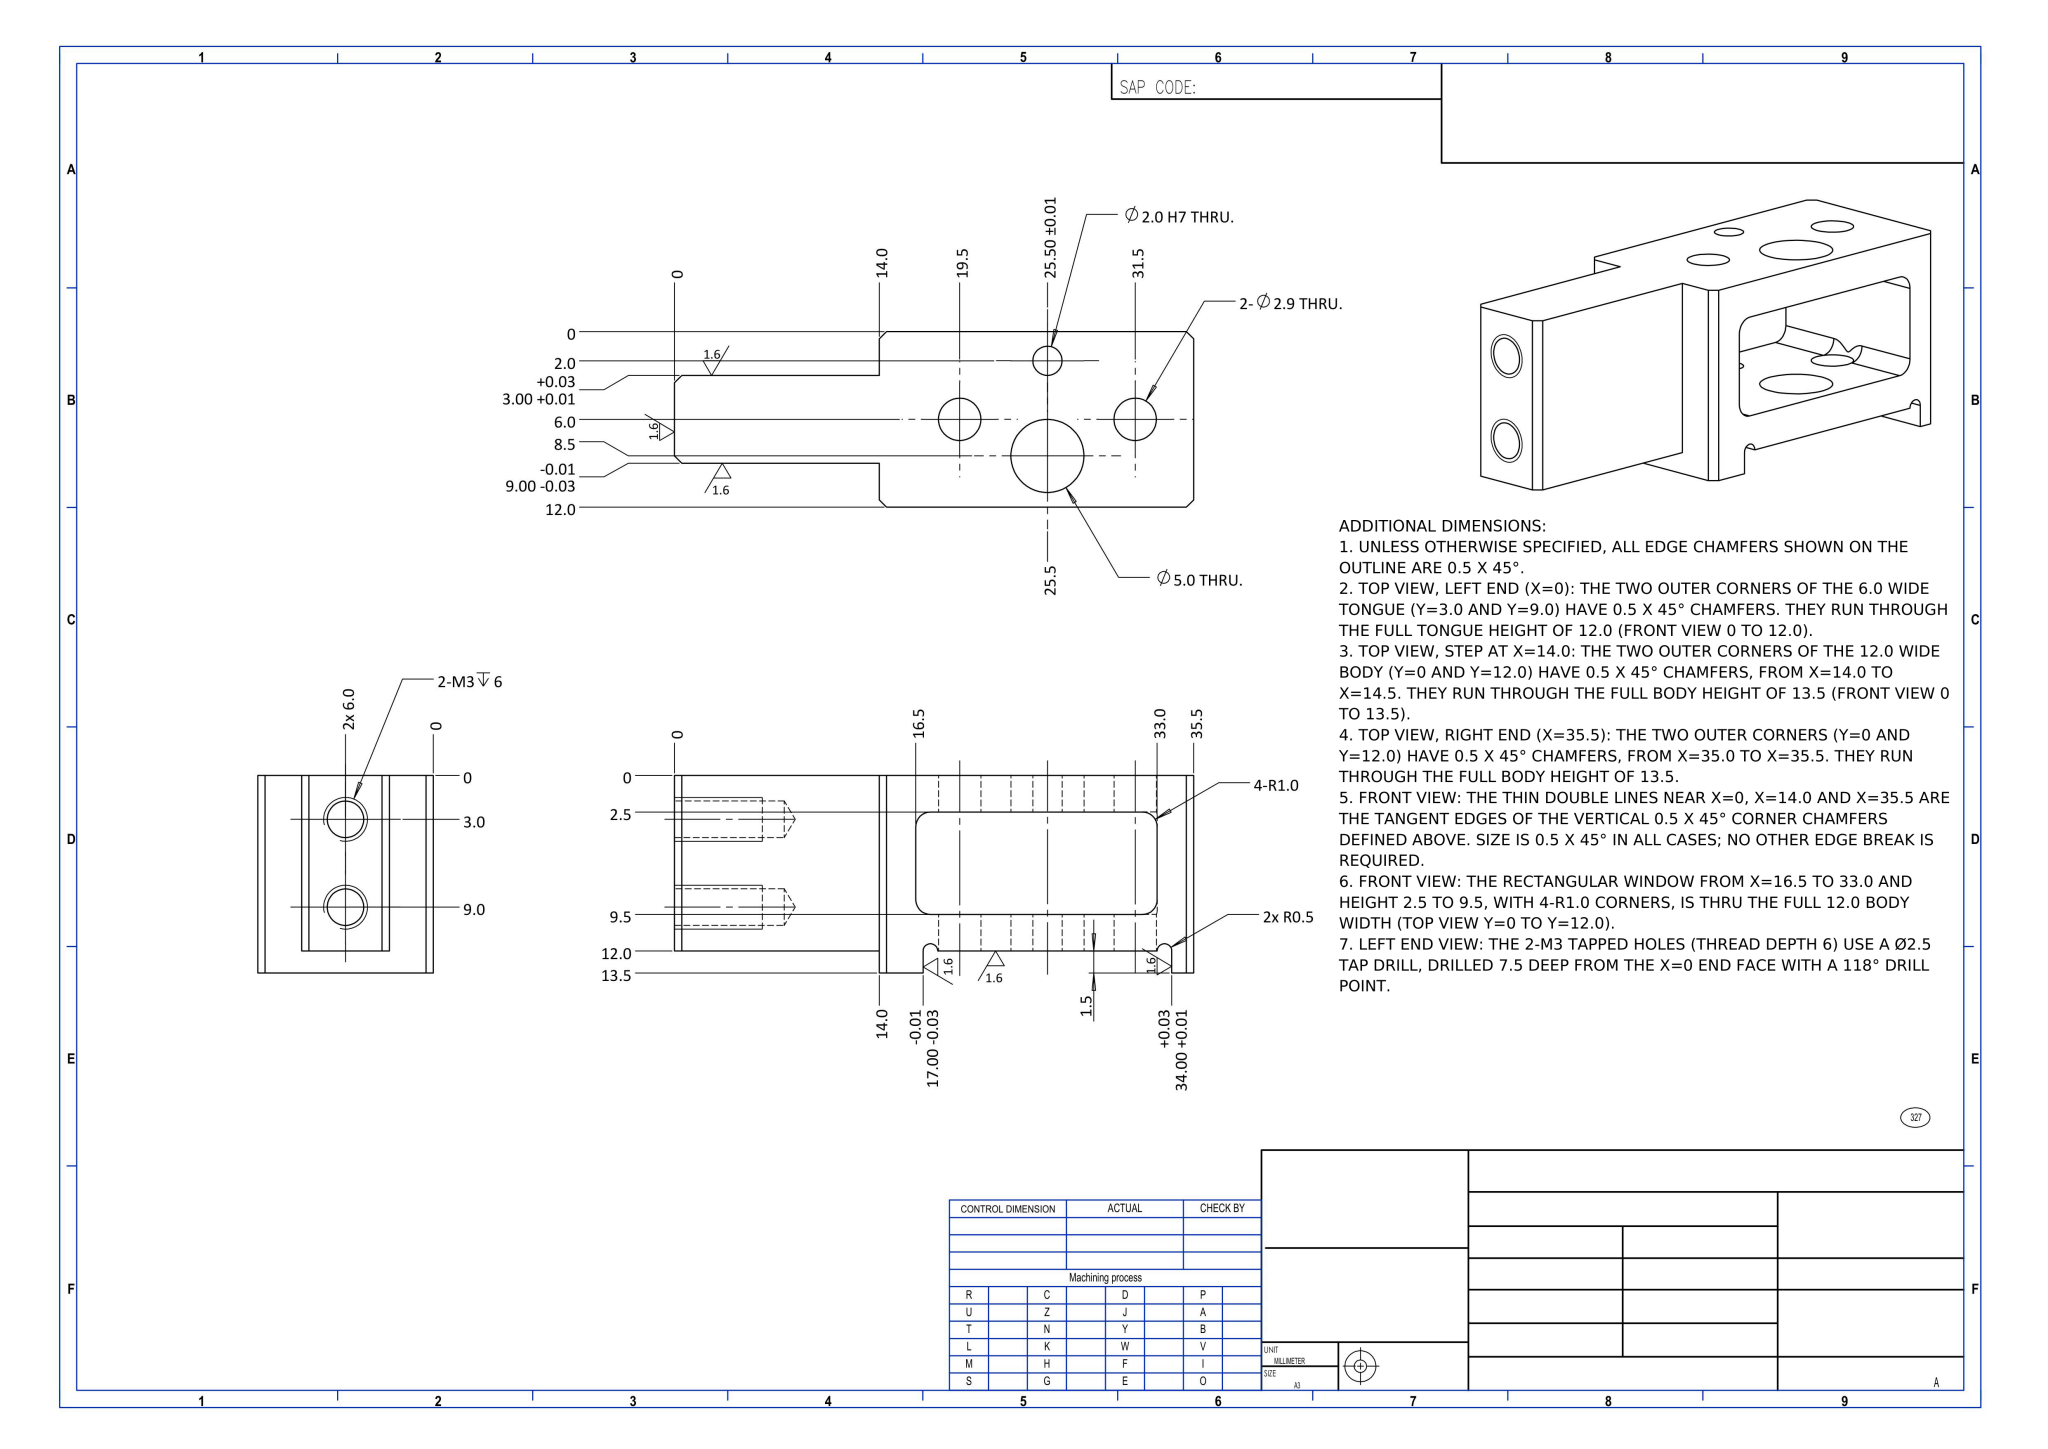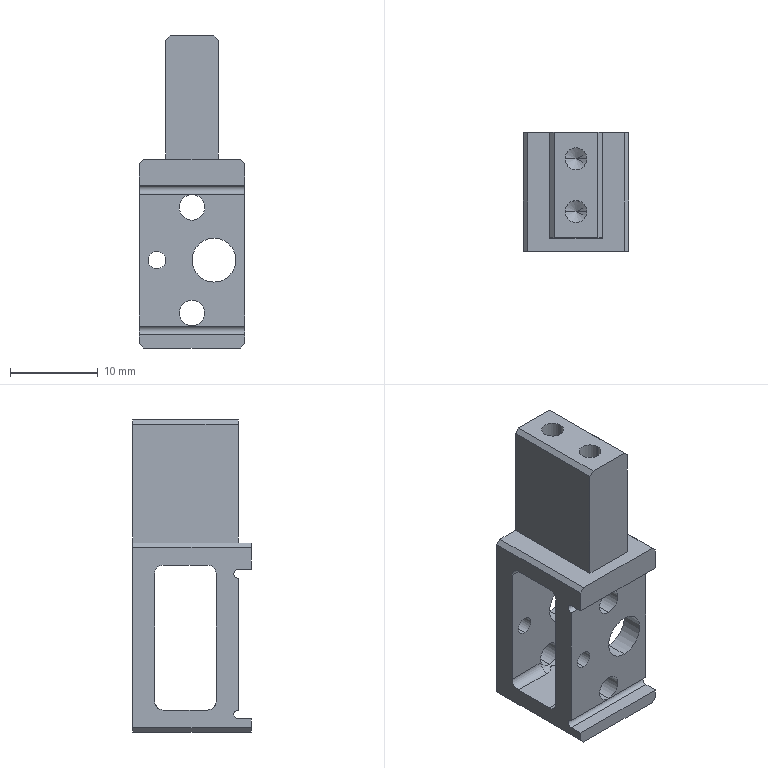Part | NX | mm | Stepped Flanged Manifold Block | 1 solid | 58 faces | box 12 x 13.5 x 35.5 mm | volume 2533 mm3 | cylinder 28 | plane 24 | cone 4 | spline 2 | commonest cylinder face diameters 2 x10 2.9 x8 2.5 x4 5 x4 1 x2